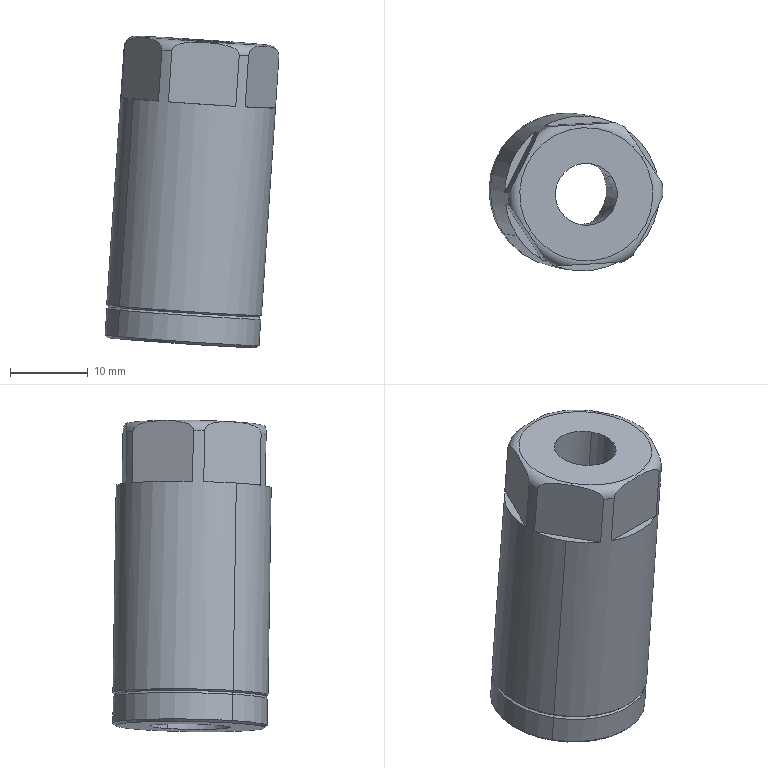Component | SolidWorks | SDAJ25x20-20B(00)+()-1_SDA-25-M8x1_2520 - A_Nut-1 | 1 solid | 33 faces | volume 8917 mm3 | plane 15 | cylinder 8 | cone 8 | torus 2 | commonest cylinder face diameters 8 x2 10.5 x2 19.9 x2 20 x2